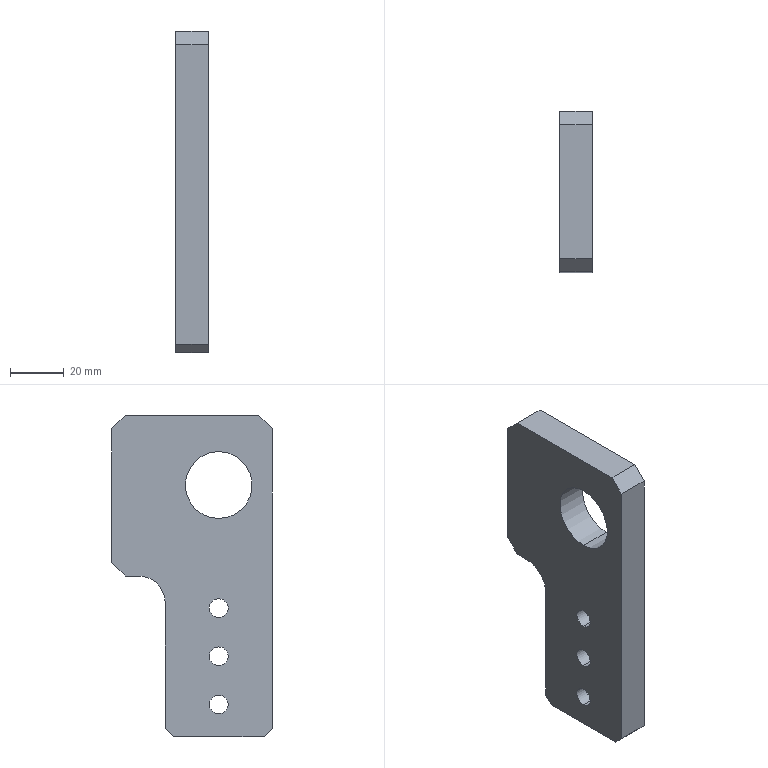Component | SolidWorks | ConveyorMotorFixingPlate-1 | 1 solid | 22 faces | box 12 x 60 x 120 mm | volume 64424 mm3 | plane 13 | cylinder 9 | commonest cylinder face diameters 7 x6 25 x2 20 x1 | material Plain Carbon Steel
build123d program:
from build123d import *

# Parameters (mm, degrees)
BOSS_EXTRUDE1_DEPTH = 12
SKETCH2_R           = 12.5
CUT_EXTRUDE1_DEPTH  = 74.103
SKETCH3_R           = 3.5
CUT_EXTRUDE2_DEPTH  = 74.103
FILLET1_R           = 10
CHAMFER1_SIZE       = 5
CHAMFER2_SIZE       = 3


with BuildPart() as part:
    # Sketch1 → Boss-Extrude1 (new body)
    with BuildSketch(Plane(origin=(0, 0, 0), x_dir=(0, 0, -1), z_dir=(1, 0, 0))):
        Polygon((0, 20), (0, 40), (60, 40), (60, 20), (60, -20), (-60, -20), (-60, 20), align=None)
    extrude(amount=BOSS_EXTRUDE1_DEPTH)

    # Sketch2 → Cut-Extrude1 (cut, through all)
    with BuildSketch(Plane(origin=(12, 0, 0), x_dir=(0, 0, -1), z_dir=(1, 0, 0))):
        with Locations((34, 0)):
            Circle(SKETCH2_R)
    extrude(amount=-CUT_EXTRUDE1_DEPTH, mode=Mode.SUBTRACT)

    # Sketch3 → Cut-Extrude2 (cut, through all)
    with BuildSketch(Plane.ZY):
        with Locations((48, 0)):
            Circle(SKETCH3_R)
        with Locations((12, 0)):
            Circle(SKETCH3_R)
        with Locations((30, 0)):
            Circle(SKETCH3_R)
    extrude(amount=-CUT_EXTRUDE2_DEPTH, mode=Mode.SUBTRACT)

    # Fillet1
    fillet1_edges = [part.edges().sort_by_distance(p)[0] for p in [
        (6, 20, 0),
    ]]
    fillet(fillet1_edges, radius=FILLET1_R)

    # Chamfer1
    chamfer1_edges = [part.edges().sort_by_distance(p)[0] for p in [
        (6, -20, -60),
        (6, 40, 0),
        (6, 40, -60),
    ]]
    chamfer(chamfer1_edges, length=CHAMFER1_SIZE)

    # Chamfer2
    chamfer2_edges = [part.edges().sort_by_distance(p)[0] for p in [
        (6, -20, 60),
        (6, 20, 60),
    ]]
    chamfer(chamfer2_edges, length=CHAMFER2_SIZE)


solid = part.part

# Placed as in the assembly
solid = solid.moved(Location((-44.55, 5.646, 1501), (-180, 0, 180)))
STEP:
#1=COLOUR_RGB('',0.7922,0.8196,0.9333);
#2=FILL_AREA_STYLE_COLOUR('',#1);
#3=FILL_AREA_STYLE('',(#2));
#4=SURFACE_STYLE_FILL_AREA(#3);
#5=SURFACE_SIDE_STYLE('',(#4));
#6=SURFACE_STYLE_USAGE(.BOTH.,#5);
#7=PRESENTATION_STYLE_ASSIGNMENT((#6));
#8=CARTESIAN_POINT('',(-2.226,0.2223,58.051));
#9=VERTEX_POINT('',#8);
#10=CARTESIAN_POINT('',(-2.226,0.2223,57.776));
#11=VERTEX_POINT('',#10);
#12=CARTESIAN_POINT('',(-2.226,0.2223,57.913));
#13=DIRECTION('',(1.,-0.,-0.));
#14=DIRECTION('',(0.,0.,-1.));
#15=AXIS2_PLACEMENT_3D('',#12,#13,#14);
#16=CIRCLE('',#15,0.1378);
#17=EDGE_CURVE('',#9,#11,#16,.T.);
#18=ORIENTED_EDGE('',*,*,#17,.F.);
#19=CARTESIAN_POINT('',(-1.754,0.2223,58.051));
#20=VERTEX_POINT('',#19);
#21=CARTESIAN_POINT('',(-2.226,0.2223,58.051));
#22=DIRECTION('',(1.,-0.,-0.));
#23=VECTOR('',#22,39.37);
#24=LINE('',#21,#23);
#25=EDGE_CURVE('',#9,#20,#24,.T.);
#26=ORIENTED_EDGE('',*,*,#25,.T.);
#27=CARTESIAN_POINT('',(-1.754,0.2223,57.776));
#28=VERTEX_POINT('',#27);
#29=CARTESIAN_POINT('',(-1.754,0.2223,57.913));
#30=DIRECTION('',(1.,-0.,-0.));
#31=DIRECTION('',(0.,0.,-1.));
#32=AXIS2_PLACEMENT_3D('',#29,#30,#31);
#33=CIRCLE('',#32,0.1378);
#34=EDGE_CURVE('',#20,#28,#33,.T.);
#35=ORIENTED_EDGE('',*,*,#34,.T.);
#36=CARTESIAN_POINT('',(-2.226,0.2223,57.776));
#37=DIRECTION('',(1.,-0.,-0.));
#38=VECTOR('',#37,39.37);
#39=LINE('',#36,#38);
#40=EDGE_CURVE('',#11,#28,#39,.T.);
#41=ORIENTED_EDGE('',*,*,#40,.F.);
#42=EDGE_LOOP('',(#18,#26,#35,#41));
#43=FACE_OUTER_BOUND('',#42,.T.);
#44=CARTESIAN_POINT('',(-2.226,0.2223,57.913));
#45=DIRECTION('',(1.,-0.,-0.));
#46=DIRECTION('',(0.,0.,-1.));
#47=AXIS2_PLACEMENT_3D('',#44,#45,#46);
#48=CYLINDRICAL_SURFACE('',#47,0.1378);
#49=ADVANCED_FACE('',(#43),#48,.F.);
#50=CARTESIAN_POINT('',(-2.226,0.2223,58.76));
#51=VERTEX_POINT('',#50);
#52=CARTESIAN_POINT('',(-2.226,0.2223,58.484));
#53=VERTEX_POINT('',#52);
#54=CARTESIAN_POINT('',(-2.226,0.2223,58.622));
#55=DIRECTION('',(1.,-0.,-0.));
#56=DIRECTION('',(0.,0.,-1.));
#57=AXIS2_PLACEMENT_3D('',#54,#55,#56);
#58=CIRCLE('',#57,0.1378);
#59=EDGE_CURVE('',#51,#53,#58,.T.);
#60=ORIENTED_EDGE('',*,*,#59,.F.);
#61=CARTESIAN_POINT('',(-1.754,0.2223,58.76));
#62=VERTEX_POINT('',#61);
#63=CARTESIAN_POINT('',(-2.226,0.2223,58.76));
#64=DIRECTION('',(1.,-0.,-0.));
#65=VECTOR('',#64,39.37);
#66=LINE('',#63,#65);
#67=EDGE_CURVE('',#51,#62,#66,.T.);
#68=ORIENTED_EDGE('',*,*,#67,.T.);
#69=CARTESIAN_POINT('',(-1.754,0.2223,58.484));
#70=VERTEX_POINT('',#69);
#71=CARTESIAN_POINT('',(-1.754,0.2223,58.622));
#72=DIRECTION('',(1.,-0.,-0.));
#73=DIRECTION('',(0.,0.,-1.));
#74=AXIS2_PLACEMENT_3D('',#71,#72,#73);
#75=CIRCLE('',#74,0.1378);
#76=EDGE_CURVE('',#62,#70,#75,.T.);
#77=ORIENTED_EDGE('',*,*,#76,.T.);
#78=CARTESIAN_POINT('',(-2.226,0.2223,58.484));
#79=DIRECTION('',(1.,-0.,-0.));
#80=VECTOR('',#79,39.37);
#81=LINE('',#78,#80);
#82=EDGE_CURVE('',#53,#70,#81,.T.);
#83=ORIENTED_EDGE('',*,*,#82,.F.);
#84=EDGE_LOOP('',(#60,#68,#77,#83));
#85=FACE_OUTER_BOUND('',#84,.T.);
#86=CARTESIAN_POINT('',(-2.226,0.2223,58.622));
#87=DIRECTION('',(1.,-0.,-0.));
#88=DIRECTION('',(0.,0.,-1.));
#89=AXIS2_PLACEMENT_3D('',#86,#87,#88);
#90=CYLINDRICAL_SURFACE('',#89,0.1378);
#91=ADVANCED_FACE('',(#85),#90,.F.);
#92=CARTESIAN_POINT('',(-2.226,0.2223,57.343));
#93=VERTEX_POINT('',#92);
#94=CARTESIAN_POINT('',(-2.226,0.2223,57.067));
#95=VERTEX_POINT('',#94);
#96=CARTESIAN_POINT('',(-2.226,0.2223,57.205));
#97=DIRECTION('',(1.,-0.,-0.));
#98=DIRECTION('',(0.,0.,-1.));
#99=AXIS2_PLACEMENT_3D('',#96,#97,#98);
#100=CIRCLE('',#99,0.1378);
#101=EDGE_CURVE('',#93,#95,#100,.T.);
#102=ORIENTED_EDGE('',*,*,#101,.F.);
#103=CARTESIAN_POINT('',(-1.754,0.2223,57.343));
#104=VERTEX_POINT('',#103);
#105=CARTESIAN_POINT('',(-2.226,0.2223,57.343));
#106=DIRECTION('',(1.,-0.,-0.));
#107=VECTOR('',#106,39.37);
#108=LINE('',#105,#107);
#109=EDGE_CURVE('',#93,#104,#108,.T.);
#110=ORIENTED_EDGE('',*,*,#109,.T.);
#111=CARTESIAN_POINT('',(-1.754,0.2223,57.067));
#112=VERTEX_POINT('',#111);
#113=CARTESIAN_POINT('',(-1.754,0.2223,57.205));
#114=DIRECTION('',(1.,-0.,-0.));
#115=DIRECTION('',(0.,0.,-1.));
#116=AXIS2_PLACEMENT_3D('',#113,#114,#115);
#117=CIRCLE('',#116,0.1378);
#118=EDGE_CURVE('',#104,#112,#117,.T.);
#119=ORIENTED_EDGE('',*,*,#118,.T.);
#120=CARTESIAN_POINT('',(-2.226,0.2223,57.067));
#121=DIRECTION('',(1.,-0.,-0.));
#122=VECTOR('',#121,39.37);
#123=LINE('',#120,#122);
#124=EDGE_CURVE('',#95,#112,#123,.T.);
#125=ORIENTED_EDGE('',*,*,#124,.F.);
#126=EDGE_LOOP('',(#102,#110,#119,#125));
#127=FACE_OUTER_BOUND('',#126,.T.);
#128=CARTESIAN_POINT('',(-2.226,0.2223,57.205));
#129=DIRECTION('',(1.,-0.,-0.));
#130=DIRECTION('',(0.,0.,-1.));
#131=AXIS2_PLACEMENT_3D('',#128,#129,#130);
#132=CYLINDRICAL_SURFACE('',#131,0.1378);
#133=ADVANCED_FACE('',(#127),#132,.F.);
#134=CARTESIAN_POINT('',(-1.754,0.2223,59.941));
#135=VERTEX_POINT('',#134);
#136=CARTESIAN_POINT('',(-1.754,0.2223,60.925));
#137=VERTEX_POINT('',#136);
#138=CARTESIAN_POINT('',(-1.754,0.2223,60.433));
#139=DIRECTION('',(-1.,0.,0.));
#140=DIRECTION('',(0.,-0.,1.));
#141=AXIS2_PLACEMENT_3D('',#138,#139,#140);
#142=CIRCLE('',#141,0.4921);
#143=EDGE_CURVE('',#135,#137,#142,.T.);
#144=ORIENTED_EDGE('',*,*,#143,.F.);
#145=CARTESIAN_POINT('',(-2.226,0.2223,59.941));
#146=VERTEX_POINT('',#145);
#147=CARTESIAN_POINT('',(-1.754,0.2223,59.941));
#148=DIRECTION('',(-1.,0.,0.));
#149=VECTOR('',#148,39.37);
#150=LINE('',#147,#149);
#151=EDGE_CURVE('',#135,#146,#150,.T.);
#152=ORIENTED_EDGE('',*,*,#151,.T.);
#153=CARTESIAN_POINT('',(-2.226,0.2223,60.925));
#154=VERTEX_POINT('',#153);
#155=CARTESIAN_POINT('',(-2.226,0.2223,60.433));
#156=DIRECTION('',(-1.,0.,0.));
#157=DIRECTION('',(0.,-0.,1.));
#158=AXIS2_PLACEMENT_3D('',#155,#156,#157);
#159=CIRCLE('',#158,0.4921);
#160=EDGE_CURVE('',#146,#154,#159,.T.);
#161=ORIENTED_EDGE('',*,*,#160,.T.);
#162=CARTESIAN_POINT('',(-1.754,0.2223,60.925));
#163=DIRECTION('',(-1.,0.,0.));
#164=VECTOR('',#163,39.37);
#165=LINE('',#162,#164);
#166=EDGE_CURVE('',#137,#154,#165,.T.);
#167=ORIENTED_EDGE('',*,*,#166,.F.);
#168=EDGE_LOOP('',(#144,#152,#161,#167));
#169=FACE_OUTER_BOUND('',#168,.T.);
#170=CARTESIAN_POINT('',(-1.754,0.2223,60.433));
#171=DIRECTION('',(-1.,0.,0.));
#172=DIRECTION('',(0.,-0.,1.));
#173=AXIS2_PLACEMENT_3D('',#170,#171,#172);
#174=CYLINDRICAL_SURFACE('',#173,0.4921);
#175=ADVANCED_FACE('',(#169),#174,.F.);
#176=CARTESIAN_POINT('',(-2.226,1.797,61.26));
#177=VERTEX_POINT('',#176);
#178=CARTESIAN_POINT('',(-2.226,1.797,59.291));
#179=VERTEX_POINT('',#178);
#180=CARTESIAN_POINT('',(-2.226,1.797,59.094));
#181=DIRECTION('',(-0.,0.,-1.));
#182=VECTOR('',#181,39.37);
#183=LINE('',#180,#182);
#184=EDGE_CURVE('',#177,#179,#183,.T.);
#185=ORIENTED_EDGE('',*,*,#184,.F.);
#186=CARTESIAN_POINT('',(-1.754,1.797,61.26));
#187=VERTEX_POINT('',#186);
#188=CARTESIAN_POINT('',(-2.226,1.797,61.26));
#189=DIRECTION('',(1.,-0.,-0.));
#190=VECTOR('',#189,39.37);
#191=LINE('',#188,#190);
#192=EDGE_CURVE('',#177,#187,#191,.T.);
#193=ORIENTED_EDGE('',*,*,#192,.T.);
#194=CARTESIAN_POINT('',(-1.754,1.797,59.291));
#195=VERTEX_POINT('',#194);
#196=CARTESIAN_POINT('',(-1.754,1.797,59.094));
#197=DIRECTION('',(-0.,0.,-1.));
#198=VECTOR('',#197,39.37);
#199=LINE('',#196,#198);
#200=EDGE_CURVE('',#187,#195,#199,.T.);
#201=ORIENTED_EDGE('',*,*,#200,.T.);
#202=CARTESIAN_POINT('',(-2.226,1.797,59.291));
#203=DIRECTION('',(-1.,0.,0.));
#204=VECTOR('',#203,39.37);
#205=LINE('',#202,#204);
#206=EDGE_CURVE('',#195,#179,#205,.T.);
#207=ORIENTED_EDGE('',*,*,#206,.T.);
#208=EDGE_LOOP('',(#185,#193,#201,#207));
#209=FACE_OUTER_BOUND('',#208,.T.);
#210=CARTESIAN_POINT('',(-2.226,1.797,59.094));
#211=DIRECTION('',(0.,-1.,-0.));
#212=DIRECTION('',(0.,-0.,1.));
#213=AXIS2_PLACEMENT_3D('',#210,#211,#212);
#214=PLANE('',#213);
#215=ADVANCED_FACE('',(#209),#214,.F.);
#216=CARTESIAN_POINT('',(-2.226,1.6,59.094));
#217=VERTEX_POINT('',#216);
#218=CARTESIAN_POINT('',(-2.226,1.403,59.094));
#219=VERTEX_POINT('',#218);
#220=CARTESIAN_POINT('',(-2.226,1.01,59.094));
#221=DIRECTION('',(0.,-1.,-0.));
#222=VECTOR('',#221,39.37);
#223=LINE('',#220,#222);
#224=EDGE_CURVE('',#217,#219,#223,.T.);
#225=ORIENTED_EDGE('',*,*,#224,.F.);
#226=CARTESIAN_POINT('',(-1.754,1.6,59.094));
#227=VERTEX_POINT('',#226);
#228=CARTESIAN_POINT('',(-2.226,1.6,59.094));
#229=DIRECTION('',(1.,-0.,-0.));
#230=VECTOR('',#229,39.37);
#231=LINE('',#228,#230);
#232=EDGE_CURVE('',#217,#227,#231,.T.);
#233=ORIENTED_EDGE('',*,*,#232,.T.);
#234=CARTESIAN_POINT('',(-1.754,1.403,59.094));
#235=VERTEX_POINT('',#234);
#236=CARTESIAN_POINT('',(-1.754,1.01,59.094));
#237=DIRECTION('',(0.,-1.,-0.));
#238=VECTOR('',#237,39.37);
#239=LINE('',#236,#238);
#240=EDGE_CURVE('',#227,#235,#239,.T.);
#241=ORIENTED_EDGE('',*,*,#240,.T.);
#242=CARTESIAN_POINT('',(-2.226,1.403,59.094));
#243=DIRECTION('',(-1.,0.,0.));
#244=VECTOR('',#243,39.37);
#245=LINE('',#242,#244);
#246=EDGE_CURVE('',#235,#219,#245,.T.);
#247=ORIENTED_EDGE('',*,*,#246,.T.);
#248=EDGE_LOOP('',(#225,#233,#241,#247));
#249=FACE_OUTER_BOUND('',#248,.T.);
#250=CARTESIAN_POINT('',(-2.226,1.01,59.094));
#251=DIRECTION('',(0.,-0.,1.));
#252=DIRECTION('',(-0.,1.,0.));
#253=AXIS2_PLACEMENT_3D('',#250,#251,#252);
#254=PLANE('',#253);
#255=ADVANCED_FACE('',(#249),#254,.F.);
#256=CARTESIAN_POINT('',(-1.754,1.01,58.701));
#257=VERTEX_POINT('',#256);
#258=CARTESIAN_POINT('',(-1.754,1.01,56.85));
#259=VERTEX_POINT('',#258);
#260=CARTESIAN_POINT('',(-1.754,1.01,56.732));
#261=DIRECTION('',(-0.,0.,-1.));
#262=VECTOR('',#261,39.37);
#263=LINE('',#260,#262);
#264=EDGE_CURVE('',#257,#259,#263,.T.);
#265=ORIENTED_EDGE('',*,*,#264,.T.);
#266=CARTESIAN_POINT('',(-2.226,1.01,56.85));
#267=VERTEX_POINT('',#266);
#268=CARTESIAN_POINT('',(-2.226,1.01,56.85));
#269=DIRECTION('',(-1.,0.,0.));
#270=VECTOR('',#269,39.37);
#271=LINE('',#268,#270);
#272=EDGE_CURVE('',#259,#267,#271,.T.);
#273=ORIENTED_EDGE('',*,*,#272,.T.);
#274=CARTESIAN_POINT('',(-2.226,1.01,58.701));
#275=VERTEX_POINT('',#274);
#276=CARTESIAN_POINT('',(-2.226,1.01,56.732));
#277=DIRECTION('',(-0.,0.,-1.));
#278=VECTOR('',#277,39.37);
#279=LINE('',#276,#278);
#280=EDGE_CURVE('',#275,#267,#279,.T.);
#281=ORIENTED_EDGE('',*,*,#280,.F.);
#282=CARTESIAN_POINT('',(-1.754,1.01,58.701));
#283=DIRECTION('',(1.,-0.,-0.));
#284=VECTOR('',#283,39.37);
#285=LINE('',#282,#284);
#286=EDGE_CURVE('',#275,#257,#285,.T.);
#287=ORIENTED_EDGE('',*,*,#286,.T.);
#288=EDGE_LOOP('',(#265,#273,#281,#287));
#289=FACE_OUTER_BOUND('',#288,.T.);
#290=CARTESIAN_POINT('',(-2.226,1.01,56.732));
#291=DIRECTION('',(0.,-1.,-0.));
#292=DIRECTION('',(0.,-0.,1.));
#293=AXIS2_PLACEMENT_3D('',#290,#291,#292);
#294=PLANE('',#293);
#295=ADVANCED_FACE('',(#289),#294,.F.);
#296=CARTESIAN_POINT('',(-1.754,0.8916,56.732));
#297=VERTEX_POINT('',#296);
#298=CARTESIAN_POINT('',(-1.754,-0.447,56.732));
#299=VERTEX_POINT('',#298);
#300=CARTESIAN_POINT('',(-1.754,-0.5651,56.732));
#301=DIRECTION('',(0.,-1.,-0.));
#302=VECTOR('',#301,39.37);
#303=LINE('',#300,#302);
#304=EDGE_CURVE('',#297,#299,#303,.T.);
#305=ORIENTED_EDGE('',*,*,#304,.T.);
#306=CARTESIAN_POINT('',(-2.226,-0.447,56.732));
#307=VERTEX_POINT('',#306);
#308=CARTESIAN_POINT('',(-2.226,-0.447,56.732));
#309=DIRECTION('',(-1.,0.,0.));
#310=VECTOR('',#309,39.37);
#311=LINE('',#308,#310);
#312=EDGE_CURVE('',#299,#307,#311,.T.);
#313=ORIENTED_EDGE('',*,*,#312,.T.);
#314=CARTESIAN_POINT('',(-2.226,0.8916,56.732));
#315=VERTEX_POINT('',#314);
#316=CARTESIAN_POINT('',(-2.226,-0.5651,56.732));
#317=DIRECTION('',(0.,-1.,-0.));
#318=VECTOR('',#317,39.37);
#319=LINE('',#316,#318);
#320=EDGE_CURVE('',#315,#307,#319,.T.);
#321=ORIENTED_EDGE('',*,*,#320,.F.);
#322=CARTESIAN_POINT('',(-2.226,0.8916,56.732));
#323=DIRECTION('',(1.,-0.,-0.));
#324=VECTOR('',#323,39.37);
#325=LINE('',#322,#324);
#326=EDGE_CURVE('',#315,#297,#325,.T.);
#327=ORIENTED_EDGE('',*,*,#326,.T.);
#328=EDGE_LOOP('',(#305,#313,#321,#327));
#329=FACE_OUTER_BOUND('',#328,.T.);
#330=CARTESIAN_POINT('',(-2.226,-0.5651,56.732));
#331=DIRECTION('',(0.,-0.,1.));
#332=DIRECTION('',(1.,-0.,-0.));
#333=AXIS2_PLACEMENT_3D('',#330,#331,#332);
#334=PLANE('',#333);
#335=ADVANCED_FACE('',(#329),#334,.F.);
#336=CARTESIAN_POINT('',(-2.226,-0.5651,56.85));
#337=VERTEX_POINT('',#336);
#338=CARTESIAN_POINT('',(-2.226,-0.5651,61.26));
#339=VERTEX_POINT('',#338);
#340=CARTESIAN_POINT('',(-2.226,-0.5651,56.732));
#341=DIRECTION('',(0.,-0.,1.));
#342=VECTOR('',#341,39.37);
#343=LINE('',#340,#342);
#344=EDGE_CURVE('',#337,#339,#343,.T.);
#345=ORIENTED_EDGE('',*,*,#344,.F.);
#346=CARTESIAN_POINT('',(-1.754,-0.5651,56.85));
#347=VERTEX_POINT('',#346);
#348=CARTESIAN_POINT('',(-2.226,-0.5651,56.85));
#349=DIRECTION('',(1.,-0.,-0.));
#350=VECTOR('',#349,39.37);
#351=LINE('',#348,#350);
#352=EDGE_CURVE('',#337,#347,#351,.T.);
#353=ORIENTED_EDGE('',*,*,#352,.T.);
#354=CARTESIAN_POINT('',(-1.754,-0.5651,61.26));
#355=VERTEX_POINT('',#354);
#356=CARTESIAN_POINT('',(-1.754,-0.5651,56.732));
#357=DIRECTION('',(0.,-0.,1.));
#358=VECTOR('',#357,39.37);
#359=LINE('',#356,#358);
#360=EDGE_CURVE('',#347,#355,#359,.T.);
#361=ORIENTED_EDGE('',*,*,#360,.T.);
#362=CARTESIAN_POINT('',(-2.226,-0.5651,61.26));
#363=DIRECTION('',(-1.,0.,0.));
#364=VECTOR('',#363,39.37);
#365=LINE('',#362,#364);
#366=EDGE_CURVE('',#355,#339,#365,.T.);
#367=ORIENTED_EDGE('',*,*,#366,.T.);
#368=EDGE_LOOP('',(#345,#353,#361,#367));
#369=FACE_OUTER_BOUND('',#368,.T.);
#370=CARTESIAN_POINT('',(-2.226,-0.5651,56.732));
#371=DIRECTION('',(-0.,1.,0.));
#372=DIRECTION('',(-0.,0.,-1.));
#373=AXIS2_PLACEMENT_3D('',#370,#371,#372);
#374=PLANE('',#373);
#375=ADVANCED_FACE('',(#369),#374,.F.);
#376=CARTESIAN_POINT('',(-2.226,-0.3683,61.457));
#377=VERTEX_POINT('',#376);
#378=CARTESIAN_POINT('',(-2.226,1.6,61.457));
#379=VERTEX_POINT('',#378);
#380=CARTESIAN_POINT('',(-2.226,1.797,61.457));
#381=DIRECTION('',(-0.,1.,0.));
#382=VECTOR('',#381,39.37);
#383=LINE('',#380,#382);
#384=EDGE_CURVE('',#377,#379,#383,.T.);
#385=ORIENTED_EDGE('',*,*,#384,.F.);
#386=CARTESIAN_POINT('',(-1.754,-0.3683,61.457));
#387=VERTEX_POINT('',#386);
#388=CARTESIAN_POINT('',(-2.226,-0.3683,61.457));
#389=DIRECTION('',(1.,-0.,-0.));
#390=VECTOR('',#389,39.37);
#391=LINE('',#388,#390);
#392=EDGE_CURVE('',#377,#387,#391,.T.);
#393=ORIENTED_EDGE('',*,*,#392,.T.);
#394=CARTESIAN_POINT('',(-1.754,1.6,61.457));
#395=VERTEX_POINT('',#394);
#396=CARTESIAN_POINT('',(-1.754,-0.5651,61.457));
#397=DIRECTION('',(-0.,1.,-0.));
#398=VECTOR('',#397,39.37);
#399=LINE('',#396,#398);
#400=EDGE_CURVE('',#387,#395,#399,.T.);
#401=ORIENTED_EDGE('',*,*,#400,.T.);
#402=CARTESIAN_POINT('',(-2.226,1.6,61.457));
#403=DIRECTION('',(-1.,0.,0.));
#404=VECTOR('',#403,39.37);
#405=LINE('',#402,#404);
#406=EDGE_CURVE('',#395,#379,#405,.T.);
#407=ORIENTED_EDGE('',*,*,#406,.T.);
#408=EDGE_LOOP('',(#385,#393,#401,#407));
#409=FACE_OUTER_BOUND('',#408,.T.);
#410=CARTESIAN_POINT('',(-2.226,-0.5651,61.457));
#411=DIRECTION('',(-0.,-0.,-1.));
#412=DIRECTION('',(0.,-1.,0.));
#413=AXIS2_PLACEMENT_3D('',#410,#411,#412);
#414=PLANE('',#413);
#415=ADVANCED_FACE('',(#409),#414,.F.);
#416=CARTESIAN_POINT('',(-2.226,0.2223,57.913));
#417=DIRECTION('',(1.,-0.,-0.));
#418=DIRECTION('',(0.,0.,-1.));
#419=AXIS2_PLACEMENT_3D('',#416,#417,#418);
#420=CIRCLE('',#419,0.1378);
#421=EDGE_CURVE('',#11,#9,#420,.T.);
#422=ORIENTED_EDGE('',*,*,#421,.T.);
#423=ORIENTED_EDGE('',*,*,#17,.T.);
#424=EDGE_LOOP('',(#422,#423));
#425=FACE_BOUND('',#424,.T.);
#426=CARTESIAN_POINT('',(-2.226,0.2223,58.622));
#427=DIRECTION('',(1.,-0.,-0.));
#428=DIRECTION('',(0.,0.,-1.));
#429=AXIS2_PLACEMENT_3D('',#426,#427,#428);
#430=CIRCLE('',#429,0.1378);
#431=EDGE_CURVE('',#53,#51,#430,.T.);
#432=ORIENTED_EDGE('',*,*,#431,.T.);
#433=ORIENTED_EDGE('',*,*,#59,.T.);
#434=EDGE_LOOP('',(#432,#433));
#435=FACE_BOUND('',#434,.T.);
#436=CARTESIAN_POINT('',(-2.226,0.2223,57.205));
#437=DIRECTION('',(1.,-0.,-0.));
#438=DIRECTION('',(0.,0.,-1.));
#439=AXIS2_PLACEMENT_3D('',#436,#437,#438);
#440=CIRCLE('',#439,0.1378);
#441=EDGE_CURVE('',#95,#93,#440,.T.);
#442=ORIENTED_EDGE('',*,*,#441,.T.);
#443=ORIENTED_EDGE('',*,*,#101,.T.);
#444=EDGE_LOOP('',(#442,#443));
#445=FACE_BOUND('',#444,.T.);
#446=CARTESIAN_POINT('',(-2.226,0.2223,60.433));
#447=DIRECTION('',(-1.,0.,0.));
#448=DIRECTION('',(0.,-0.,1.));
#449=AXIS2_PLACEMENT_3D('',#446,#447,#448);
#450=CIRCLE('',#449,0.4921);
#451=EDGE_CURVE('',#154,#146,#450,.T.);
#452=ORIENTED_EDGE('',*,*,#451,.F.);
#453=ORIENTED_EDGE('',*,*,#160,.F.);
#454=EDGE_LOOP('',(#452,#453));
#455=FACE_BOUND('',#454,.T.);
#456=ORIENTED_EDGE('',*,*,#320,.T.);
#457=CARTESIAN_POINT('',(-2.226,-1.293,57.579));
#458=DIRECTION('',(0.,-0.7071,0.7071));
#459=VECTOR('',#458,39.37);
#460=LINE('',#457,#459);
#461=EDGE_CURVE('',#307,#337,#460,.T.);
#462=ORIENTED_EDGE('',*,*,#461,.T.);
#463=ORIENTED_EDGE('',*,*,#344,.T.);
#464=CARTESIAN_POINT('',(-2.226,-1.254,60.571));
#465=DIRECTION('',(0.,0.7071,0.7071));
#466=VECTOR('',#465,39.37);
#467=LINE('',#464,#466);
#468=EDGE_CURVE('',#339,#377,#467,.T.);
#469=ORIENTED_EDGE('',*,*,#468,.T.);
#470=ORIENTED_EDGE('',*,*,#384,.T.);
#471=CARTESIAN_POINT('',(-2.226,2.092,60.965));
#472=DIRECTION('',(-0.,0.7071,-0.7071));
#473=VECTOR('',#472,39.37);
#474=LINE('',#471,#473);
#475=EDGE_CURVE('',#379,#177,#474,.T.);
#476=ORIENTED_EDGE('',*,*,#475,.T.);
#477=ORIENTED_EDGE('',*,*,#184,.T.);
#478=CARTESIAN_POINT('',(-2.226,0.9112,58.406));
#479=DIRECTION('',(-0.,-0.7071,-0.7071));
#480=VECTOR('',#479,39.37);
#481=LINE('',#478,#480);
#482=EDGE_CURVE('',#179,#217,#481,.T.);
#483=ORIENTED_EDGE('',*,*,#482,.T.);
#484=ORIENTED_EDGE('',*,*,#224,.T.);
#485=CARTESIAN_POINT('',(-2.226,1.403,58.701));
#486=DIRECTION('',(1.,-0.,-0.));
#487=DIRECTION('',(0.,0.,1.));
#488=AXIS2_PLACEMENT_3D('',#485,#486,#487);
#489=CIRCLE('',#488,0.3937);
#490=EDGE_CURVE('',#219,#275,#489,.T.);
#491=ORIENTED_EDGE('',*,*,#490,.T.);
#492=ORIENTED_EDGE('',*,*,#280,.T.);
#493=CARTESIAN_POINT('',(-2.226,1.738,57.579));
#494=DIRECTION('',(-0.,-0.7071,-0.7071));
#495=VECTOR('',#494,39.37);
#496=LINE('',#493,#495);
#497=EDGE_CURVE('',#267,#315,#496,.T.);
#498=ORIENTED_EDGE('',*,*,#497,.T.);
#499=EDGE_LOOP('',(#456,#462,#463,#469,#470,#476,#477,#483,#484,#491,#492,#498));
#500=FACE_OUTER_BOUND('',#499,.T.);
#501=CARTESIAN_POINT('',(-2.226,0.2223,59.094));
#502=DIRECTION('',(-1.,0.,0.));
#503=DIRECTION('',(0.,-0.,1.));
#504=AXIS2_PLACEMENT_3D('',#501,#502,#503);
#505=PLANE('',#504);
#506=ADVANCED_FACE('',(#425,#435,#445,#455,#500),#505,.T.);
#507=CARTESIAN_POINT('',(-1.754,0.2223,57.913));
#508=DIRECTION('',(1.,-0.,-0.));
#509=DIRECTION('',(0.,0.,-1.));
#510=AXIS2_PLACEMENT_3D('',#507,#508,#509);
#511=CIRCLE('',#510,0.1378);
#512=EDGE_CURVE('',#28,#20,#511,.T.);
#513=ORIENTED_EDGE('',*,*,#512,.F.);
#514=ORIENTED_EDGE('',*,*,#34,.F.);
#515=EDGE_LOOP('',(#513,#514));
#516=FACE_BOUND('',#515,.T.);
#517=CARTESIAN_POINT('',(-1.754,0.2223,58.622));
#518=DIRECTION('',(1.,-0.,-0.));
#519=DIRECTION('',(0.,0.,-1.));
#520=AXIS2_PLACEMENT_3D('',#517,#518,#519);
#521=CIRCLE('',#520,0.1378);
#522=EDGE_CURVE('',#70,#62,#521,.T.);
#523=ORIENTED_EDGE('',*,*,#522,.F.);
#524=ORIENTED_EDGE('',*,*,#76,.F.);
#525=EDGE_LOOP('',(#523,#524));
#526=FACE_BOUND('',#525,.T.);
#527=CARTESIAN_POINT('',(-1.754,0.2223,57.205));
#528=DIRECTION('',(1.,-0.,-0.));
#529=DIRECTION('',(0.,0.,-1.));
#530=AXIS2_PLACEMENT_3D('',#527,#528,#529);
#531=CIRCLE('',#530,0.1378);
#532=EDGE_CURVE('',#112,#104,#531,.T.);
#533=ORIENTED_EDGE('',*,*,#532,.F.);
#534=ORIENTED_EDGE('',*,*,#118,.F.);
#535=EDGE_LOOP('',(#533,#534));
#536=FACE_BOUND('',#535,.T.);
#537=CARTESIAN_POINT('',(-1.754,0.2223,60.433));
#538=DIRECTION('',(-1.,0.,0.));
#539=DIRECTION('',(0.,-0.,1.));
#540=AXIS2_PLACEMENT_3D('',#537,#538,#539);
#541=CIRCLE('',#540,0.4921);
#542=EDGE_CURVE('',#137,#135,#541,.T.);
#543=ORIENTED_EDGE('',*,*,#542,.T.);
#544=ORIENTED_EDGE('',*,*,#143,.T.);
#545=EDGE_LOOP('',(#543,#544));
#546=FACE_BOUND('',#545,.T.);
#547=ORIENTED_EDGE('',*,*,#360,.F.);
#548=CARTESIAN_POINT('',(-1.754,-0.5651,56.85));
#549=DIRECTION('',(-0.,0.7071,-0.7071));
#550=VECTOR('',#549,39.37);
#551=LINE('',#548,#550);
#552=EDGE_CURVE('',#347,#299,#551,.T.);
#553=ORIENTED_EDGE('',*,*,#552,.T.);
#554=ORIENTED_EDGE('',*,*,#304,.F.);
#555=CARTESIAN_POINT('',(-1.754,0.8916,56.732));
#556=DIRECTION('',(0.,0.7071,0.7071));
#557=VECTOR('',#556,39.37);
#558=LINE('',#555,#557);
#559=EDGE_CURVE('',#297,#259,#558,.T.);
#560=ORIENTED_EDGE('',*,*,#559,.T.);
#561=ORIENTED_EDGE('',*,*,#264,.F.);
#562=CARTESIAN_POINT('',(-1.754,1.403,58.701));
#563=DIRECTION('',(-1.,0.,0.));
#564=DIRECTION('',(0.,0.,1.));
#565=AXIS2_PLACEMENT_3D('',#562,#563,#564);
#566=CIRCLE('',#565,0.3937);
#567=EDGE_CURVE('',#257,#235,#566,.T.);
#568=ORIENTED_EDGE('',*,*,#567,.T.);
#569=ORIENTED_EDGE('',*,*,#240,.F.);
#570=CARTESIAN_POINT('',(-1.754,1.6,59.094));
#571=DIRECTION('',(0.,0.7071,0.7071));
#572=VECTOR('',#571,39.37);
#573=LINE('',#570,#572);
#574=EDGE_CURVE('',#227,#195,#573,.T.);
#575=ORIENTED_EDGE('',*,*,#574,.T.);
#576=ORIENTED_EDGE('',*,*,#200,.F.);
#577=CARTESIAN_POINT('',(-1.754,1.797,61.26));
#578=DIRECTION('',(0.,-0.7071,0.7071));
#579=VECTOR('',#578,39.37);
#580=LINE('',#577,#579);
#581=EDGE_CURVE('',#187,#395,#580,.T.);
#582=ORIENTED_EDGE('',*,*,#581,.T.);
#583=ORIENTED_EDGE('',*,*,#400,.F.);
#584=CARTESIAN_POINT('',(-1.754,-0.3683,61.457));
#585=DIRECTION('',(-0.,-0.7071,-0.7071));
#586=VECTOR('',#585,39.37);
#587=LINE('',#584,#586);
#588=EDGE_CURVE('',#387,#355,#587,.T.);
#589=ORIENTED_EDGE('',*,*,#588,.T.);
#590=EDGE_LOOP('',(#547,#553,#554,#560,#561,#568,#569,#575,#576,#582,#583,#589));
#591=FACE_OUTER_BOUND('',#590,.T.);
#592=CARTESIAN_POINT('',(-1.754,0.2223,59.094));
#593=DIRECTION('',(-1.,0.,0.));
#594=DIRECTION('',(0.,-0.,1.));
#595=AXIS2_PLACEMENT_3D('',#592,#593,#594);
#596=PLANE('',#595);
#597=ADVANCED_FACE('',(#516,#526,#536,#546,#591),#596,.F.);
#598=ORIENTED_EDGE('',*,*,#151,.F.);
#599=ORIENTED_EDGE('',*,*,#542,.F.);
#600=ORIENTED_EDGE('',*,*,#166,.T.);
#601=ORIENTED_EDGE('',*,*,#451,.T.);
#602=EDGE_LOOP('',(#598,#599,#600,#601));
#603=FACE_OUTER_BOUND('',#602,.T.);
#604=CARTESIAN_POINT('',(-1.754,0.2223,60.433));
#605=DIRECTION('',(-1.,0.,0.));
#606=DIRECTION('',(0.,-0.,1.));
#607=AXIS2_PLACEMENT_3D('',#604,#605,#606);
#608=CYLINDRICAL_SURFACE('',#607,0.4921);
#609=ADVANCED_FACE('',(#603),#608,.F.);
#610=ORIENTED_EDGE('',*,*,#109,.F.);
#611=ORIENTED_EDGE('',*,*,#441,.F.);
#612=ORIENTED_EDGE('',*,*,#124,.T.);
#613=ORIENTED_EDGE('',*,*,#532,.T.);
#614=EDGE_LOOP('',(#610,#611,#612,#613));
#615=FACE_OUTER_BOUND('',#614,.T.);
#616=CARTESIAN_POINT('',(-2.226,0.2223,57.205));
#617=DIRECTION('',(1.,-0.,-0.));
#618=DIRECTION('',(0.,0.,-1.));
#619=AXIS2_PLACEMENT_3D('',#616,#617,#618);
#620=CYLINDRICAL_SURFACE('',#619,0.1378);
#621=ADVANCED_FACE('',(#615),#620,.F.);
#622=ORIENTED_EDGE('',*,*,#67,.F.);
#623=ORIENTED_EDGE('',*,*,#431,.F.);
#624=ORIENTED_EDGE('',*,*,#82,.T.);
#625=ORIENTED_EDGE('',*,*,#522,.T.);
#626=EDGE_LOOP('',(#622,#623,#624,#625));
#627=FACE_OUTER_BOUND('',#626,.T.);
#628=CARTESIAN_POINT('',(-2.226,0.2223,58.622));
#629=DIRECTION('',(1.,-0.,-0.));
#630=DIRECTION('',(0.,0.,-1.));
#631=AXIS2_PLACEMENT_3D('',#628,#629,#630);
#632=CYLINDRICAL_SURFACE('',#631,0.1378);
#633=ADVANCED_FACE('',(#627),#632,.F.);
#634=ORIENTED_EDGE('',*,*,#25,.F.);
#635=ORIENTED_EDGE('',*,*,#421,.F.);
#636=ORIENTED_EDGE('',*,*,#40,.T.);
#637=ORIENTED_EDGE('',*,*,#512,.T.);
#638=EDGE_LOOP('',(#634,#635,#636,#637));
#639=FACE_OUTER_BOUND('',#638,.T.);
#640=CARTESIAN_POINT('',(-2.226,0.2223,57.913));
#641=DIRECTION('',(1.,-0.,-0.));
#642=DIRECTION('',(0.,0.,-1.));
#643=AXIS2_PLACEMENT_3D('',#640,#641,#642);
#644=CYLINDRICAL_SURFACE('',#643,0.1378);
#645=ADVANCED_FACE('',(#639),#644,.F.);
#646=ORIENTED_EDGE('',*,*,#490,.F.);
#647=ORIENTED_EDGE('',*,*,#246,.F.);
#648=ORIENTED_EDGE('',*,*,#567,.F.);
#649=ORIENTED_EDGE('',*,*,#286,.F.);
#650=EDGE_LOOP('',(#646,#647,#648,#649));
#651=FACE_OUTER_BOUND('',#650,.T.);
#652=CARTESIAN_POINT('',(-2.226,1.403,58.701));
#653=DIRECTION('',(-1.,0.,0.));
#654=DIRECTION('',(0.,0.,1.));
#655=AXIS2_PLACEMENT_3D('',#652,#653,#654);
#656=CYLINDRICAL_SURFACE('',#655,0.3937);
#657=ADVANCED_FACE('',(#651),#656,.F.);
#658=ORIENTED_EDGE('',*,*,#468,.F.);
#659=ORIENTED_EDGE('',*,*,#366,.F.);
#660=ORIENTED_EDGE('',*,*,#588,.F.);
#661=ORIENTED_EDGE('',*,*,#392,.F.);
#662=EDGE_LOOP('',(#658,#659,#660,#661));
#663=FACE_OUTER_BOUND('',#662,.T.);
#664=CARTESIAN_POINT('',(-2.226,-0.3683,61.457));
#665=DIRECTION('',(-0.,0.7071,-0.7071));
#666=DIRECTION('',(1.,-0.,-0.));
#667=AXIS2_PLACEMENT_3D('',#664,#665,#666);
#668=PLANE('',#667);
#669=ADVANCED_FACE('',(#663),#668,.F.);
#670=ORIENTED_EDGE('',*,*,#475,.F.);
#671=ORIENTED_EDGE('',*,*,#406,.F.);
#672=ORIENTED_EDGE('',*,*,#581,.F.);
#673=ORIENTED_EDGE('',*,*,#192,.F.);
#674=EDGE_LOOP('',(#670,#671,#672,#673));
#675=FACE_OUTER_BOUND('',#674,.T.);
#676=CARTESIAN_POINT('',(-2.226,1.797,61.26));
#677=DIRECTION('',(-0.,-0.7071,-0.7071));
#678=DIRECTION('',(1.,-0.,-0.));
#679=AXIS2_PLACEMENT_3D('',#676,#677,#678);
#680=PLANE('',#679);
#681=ADVANCED_FACE('',(#675),#680,.F.);
#682=ORIENTED_EDGE('',*,*,#482,.F.);
#683=ORIENTED_EDGE('',*,*,#206,.F.);
#684=ORIENTED_EDGE('',*,*,#574,.F.);
#685=ORIENTED_EDGE('',*,*,#232,.F.);
#686=EDGE_LOOP('',(#682,#683,#684,#685));
#687=FACE_OUTER_BOUND('',#686,.T.);
#688=CARTESIAN_POINT('',(-2.226,1.6,59.094));
#689=DIRECTION('',(0.,-0.7071,0.7071));
#690=DIRECTION('',(1.,-0.,-0.));
#691=AXIS2_PLACEMENT_3D('',#688,#689,#690);
#692=PLANE('',#691);
#693=ADVANCED_FACE('',(#687),#692,.F.);
#694=ORIENTED_EDGE('',*,*,#461,.F.);
#695=ORIENTED_EDGE('',*,*,#312,.F.);
#696=ORIENTED_EDGE('',*,*,#552,.F.);
#697=ORIENTED_EDGE('',*,*,#352,.F.);
#698=EDGE_LOOP('',(#694,#695,#696,#697));
#699=FACE_OUTER_BOUND('',#698,.T.);
#700=CARTESIAN_POINT('',(-2.226,-0.5651,56.85));
#701=DIRECTION('',(0.,0.7071,0.7071));
#702=DIRECTION('',(1.,-0.,-0.));
#703=AXIS2_PLACEMENT_3D('',#700,#701,#702);
#704=PLANE('',#703);
#705=ADVANCED_FACE('',(#699),#704,.F.);
#706=ORIENTED_EDGE('',*,*,#497,.F.);
#707=ORIENTED_EDGE('',*,*,#272,.F.);
#708=ORIENTED_EDGE('',*,*,#559,.F.);
#709=ORIENTED_EDGE('',*,*,#326,.F.);
#710=EDGE_LOOP('',(#706,#707,#708,#709));
#711=FACE_OUTER_BOUND('',#710,.T.);
#712=CARTESIAN_POINT('',(-2.226,0.8916,56.732));
#713=DIRECTION('',(0.,-0.7071,0.7071));
#714=DIRECTION('',(1.,-0.,-0.));
#715=AXIS2_PLACEMENT_3D('',#712,#713,#714);
#716=PLANE('',#715);
#717=ADVANCED_FACE('',(#711),#716,.F.);
#718=CLOSED_SHELL('',(#49,#91,#133,#175,#215,#255,#295,#335,#375,#415,#506,#597,#609,#621,#633,#645,#657,#669,#681,#693,#705,#717));
#719=MANIFOLD_SOLID_BREP('',#718);
#720=STYLED_ITEM('',(#7),#719);
#721=(LENGTH_UNIT()NAMED_UNIT(*)SI_UNIT($,.METRE.));
#722=LENGTH_MEASURE_WITH_UNIT(LENGTH_MEASURE(0.0254),#721);
#723=DIMENSIONAL_EXPONENTS(1.,0.,0.,0.,0.,0.,0.);
#724=(CONVERSION_BASED_UNIT('',#722)LENGTH_UNIT()NAMED_UNIT(#723));
#725=UNCERTAINTY_MEASURE_WITH_UNIT(LENGTH_MEASURE(0.00001),#724,'','');
#726=(NAMED_UNIT(*)PLANE_ANGLE_UNIT()SI_UNIT($,.RADIAN.));
#727=(NAMED_UNIT(*)SI_UNIT($,.STERADIAN.)SOLID_ANGLE_UNIT());
#728=(GEOMETRIC_REPRESENTATION_CONTEXT(3)GLOBAL_UNCERTAINTY_ASSIGNED_CONTEXT((#725))GLOBAL_UNIT_ASSIGNED_CONTEXT((#724,#726,#727))REPRESENTATION_CONTEXT('',''));
#729=MECHANICAL_DESIGN_GEOMETRIC_PRESENTATION_REPRESENTATION('',(#720),#728);
#730=PRESENTATION_LAYER_ASSIGNMENT('','',(#720));
#731=CARTESIAN_POINT('',(0.,0.,0.));
#732=DIRECTION('',(0.,0.,1.));
#733=DIRECTION('',(1.,0.,0.));
#734=AXIS2_PLACEMENT_3D('',#731,#732,#733);
#735=(LENGTH_UNIT()NAMED_UNIT(*)SI_UNIT($,.METRE.));
#736=LENGTH_MEASURE_WITH_UNIT(LENGTH_MEASURE(0.0254),#735);
#737=DIMENSIONAL_EXPONENTS(1.,0.,0.,0.,0.,0.,0.);
#738=(CONVERSION_BASED_UNIT('',#736)LENGTH_UNIT()NAMED_UNIT(#737));
#739=UNCERTAINTY_MEASURE_WITH_UNIT(LENGTH_MEASURE(0.00001),#738,'','');
#740=(NAMED_UNIT(*)PLANE_ANGLE_UNIT()SI_UNIT($,.RADIAN.));
#741=(NAMED_UNIT(*)SI_UNIT($,.STERADIAN.)SOLID_ANGLE_UNIT());
#742=(GEOMETRIC_REPRESENTATION_CONTEXT(3)GLOBAL_UNCERTAINTY_ASSIGNED_CONTEXT((#739))GLOBAL_UNIT_ASSIGNED_CONTEXT((#738,#740,#741))REPRESENTATION_CONTEXT('',''));
#743=ADVANCED_BREP_SHAPE_REPRESENTATION('',(#719,#734),#742);